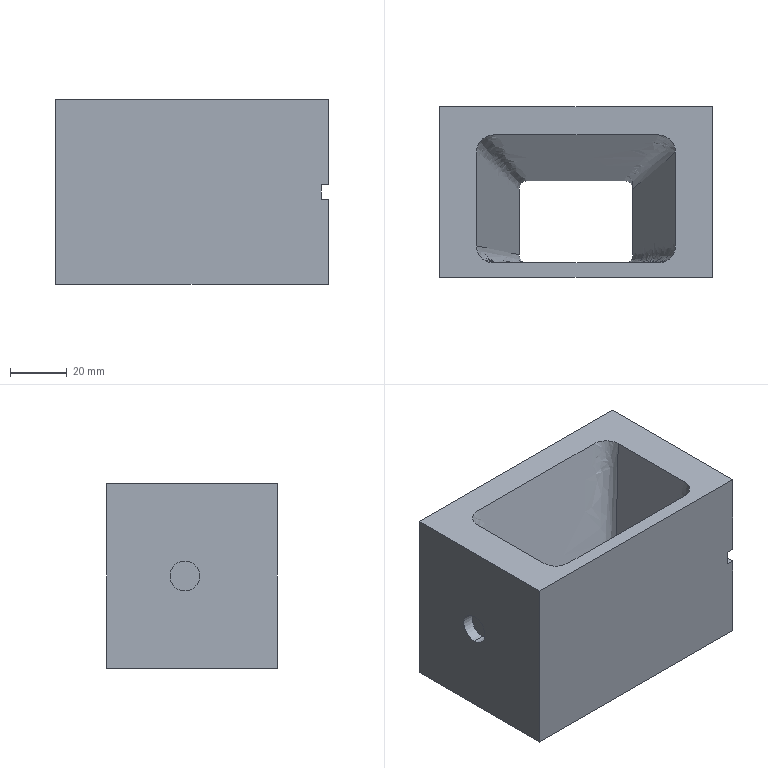Component | SolidWorks | CuttingDie-1_Mold01-1-3 | 1 solid | 15 faces | box 96 x 60 x 65 mm | volume 243310 mm3 | plane 11 | spline 2 | cylinder 2 | commonest cylinder face diameters 10.5 x2
STEP:
#1=COLOUR_RGB('',0.7922,0.8196,0.9333);
#2=FILL_AREA_STYLE_COLOUR('',#1);
#3=FILL_AREA_STYLE('',(#2));
#4=SURFACE_STYLE_FILL_AREA(#3);
#5=SURFACE_SIDE_STYLE('',(#4));
#6=SURFACE_STYLE_USAGE(.BOTH.,#5);
#7=PRESENTATION_STYLE_ASSIGNMENT((#6));
#8=CARTESIAN_POINT('',(-18.672,-11.644,44.764));
#9=VERTEX_POINT('',#8);
#10=CARTESIAN_POINT('',(-18.672,-10.345,44.764));
#11=VERTEX_POINT('',#10);
#12=CARTESIAN_POINT('',(-18.672,-10.345,44.764));
#13=DIRECTION('',(-0.,1.,0.));
#14=VECTOR('',#13,39.37);
#15=LINE('',#12,#14);
#16=EDGE_CURVE('',#9,#11,#15,.T.);
#17=ORIENTED_EDGE('',*,*,#16,.F.);
#18=CARTESIAN_POINT('',(-18.082,-11.762,42.205));
#19=VERTEX_POINT('',#18);
#20=CARTESIAN_POINT('',(-18.672,-11.644,44.764));
#21=CARTESIAN_POINT('',(-18.475,-11.684,43.911));
#22=CARTESIAN_POINT('',(-18.278,-11.723,43.058));
#23=CARTESIAN_POINT('',(-18.082,-11.762,42.205));
#24=B_SPLINE_CURVE_WITH_KNOTS('',3,(#20,#21,#22,#23),.UNSPECIFIED.,.F.,.F.,(4,4),(0.,1.),.UNSPECIFIED.);
#25=EDGE_CURVE('',#9,#19,#24,.T.);
#26=ORIENTED_EDGE('',*,*,#25,.T.);
#27=CARTESIAN_POINT('',(-18.082,-10.857,42.205));
#28=VERTEX_POINT('',#27);
#29=CARTESIAN_POINT('',(-18.082,-11.762,42.205));
#30=DIRECTION('',(0.,-1.,-0.));
#31=VECTOR('',#30,39.37);
#32=LINE('',#29,#31);
#33=EDGE_CURVE('',#28,#19,#32,.T.);
#34=ORIENTED_EDGE('',*,*,#33,.F.);
#35=CARTESIAN_POINT('',(-17.963,-10.739,42.205));
#36=VERTEX_POINT('',#35);
#37=CARTESIAN_POINT('',(-17.963,-10.857,42.205));
#38=DIRECTION('',(-0.,-0.,1.));
#39=DIRECTION('',(-1.,0.,0.));
#40=AXIS2_PLACEMENT_3D('',#37,#38,#39);
#41=CIRCLE('',#40,0.1181);
#42=EDGE_CURVE('',#36,#28,#41,.T.);
#43=ORIENTED_EDGE('',*,*,#42,.F.);
#44=CARTESIAN_POINT('',(-16.625,-10.739,42.205));
#45=VERTEX_POINT('',#44);
#46=CARTESIAN_POINT('',(-17.963,-10.739,42.205));
#47=DIRECTION('',(-1.,-0.,-0.));
#48=VECTOR('',#47,39.37);
#49=LINE('',#46,#48);
#50=EDGE_CURVE('',#45,#36,#49,.T.);
#51=ORIENTED_EDGE('',*,*,#50,.F.);
#52=CARTESIAN_POINT('',(-16.507,-10.857,42.205));
#53=VERTEX_POINT('',#52);
#54=CARTESIAN_POINT('',(-16.625,-10.857,42.205));
#55=DIRECTION('',(-0.,-0.,1.));
#56=DIRECTION('',(-1.,0.,0.));
#57=AXIS2_PLACEMENT_3D('',#54,#55,#56);
#58=CIRCLE('',#57,0.1181);
#59=EDGE_CURVE('',#53,#45,#58,.T.);
#60=ORIENTED_EDGE('',*,*,#59,.F.);
#61=CARTESIAN_POINT('',(-15.916,-10.345,44.764));
#62=VERTEX_POINT('',#61);
#63=CARTESIAN_POINT('',(-15.916,-10.345,44.764));
#64=CARTESIAN_POINT('',(-16.113,-10.516,43.911));
#65=CARTESIAN_POINT('',(-16.31,-10.686,43.058));
#66=CARTESIAN_POINT('',(-16.507,-10.857,42.205));
#67=B_SPLINE_CURVE_WITH_KNOTS('',3,(#63,#64,#65,#66),.UNSPECIFIED.,.F.,.F.,(4,4),(0.,1.),.UNSPECIFIED.);
#68=EDGE_CURVE('',#62,#53,#67,.T.);
#69=ORIENTED_EDGE('',*,*,#68,.F.);
#70=CARTESIAN_POINT('',(-16.152,-10.109,44.764));
#71=VERTEX_POINT('',#70);
#72=CARTESIAN_POINT('',(-16.152,-10.345,44.764));
#73=DIRECTION('',(0.,0.,-1.));
#74=DIRECTION('',(-1.,0.,0.));
#75=AXIS2_PLACEMENT_3D('',#72,#73,#74);
#76=CIRCLE('',#75,0.2362);
#77=EDGE_CURVE('',#71,#62,#76,.T.);
#78=ORIENTED_EDGE('',*,*,#77,.F.);
#79=CARTESIAN_POINT('',(-18.436,-10.109,44.764));
#80=VERTEX_POINT('',#79);
#81=CARTESIAN_POINT('',(-16.152,-10.109,44.764));
#82=DIRECTION('',(1.,0.,0.));
#83=VECTOR('',#82,39.37);
#84=LINE('',#81,#83);
#85=EDGE_CURVE('',#80,#71,#84,.T.);
#86=ORIENTED_EDGE('',*,*,#85,.F.);
#87=CARTESIAN_POINT('',(-18.436,-10.345,44.764));
#88=DIRECTION('',(0.,0.,-1.));
#89=DIRECTION('',(1.,0.,0.));
#90=AXIS2_PLACEMENT_3D('',#87,#88,#89);
#91=CIRCLE('',#90,0.2362);
#92=EDGE_CURVE('',#11,#80,#91,.T.);
#93=ORIENTED_EDGE('',*,*,#92,.F.);
#94=EDGE_LOOP('',(#17,#26,#34,#43,#51,#60,#69,#78,#86,#93));
#95=FACE_OUTER_BOUND('',#94,.T.);
#96=CARTESIAN_POINT('',(-15.916,-10.345,44.764));
#97=CARTESIAN_POINT('',(-16.113,-10.516,43.911));
#98=CARTESIAN_POINT('',(-16.31,-10.686,43.058));
#99=CARTESIAN_POINT('',(-16.507,-10.857,42.205));
#100=CARTESIAN_POINT('',(-15.916,-10.457,44.764));
#101=CARTESIAN_POINT('',(-16.113,-10.615,43.911));
#102=CARTESIAN_POINT('',(-16.31,-10.772,43.058));
#103=CARTESIAN_POINT('',(-16.507,-10.93,42.205));
#104=CARTESIAN_POINT('',(-15.916,-10.675,44.764));
#105=CARTESIAN_POINT('',(-16.113,-10.81,43.911));
#106=CARTESIAN_POINT('',(-16.31,-10.945,43.058));
#107=CARTESIAN_POINT('',(-16.507,-11.08,42.205));
#108=CARTESIAN_POINT('',(-15.916,-10.995,44.764));
#109=CARTESIAN_POINT('',(-16.113,-11.1,43.911));
#110=CARTESIAN_POINT('',(-16.31,-11.205,43.058));
#111=CARTESIAN_POINT('',(-16.507,-11.31,42.205));
#112=CARTESIAN_POINT('',(-15.916,-11.314,44.764));
#113=CARTESIAN_POINT('',(-16.113,-11.389,43.911));
#114=CARTESIAN_POINT('',(-16.31,-11.464,43.058));
#115=CARTESIAN_POINT('',(-16.507,-11.54,42.205));
#116=CARTESIAN_POINT('',(-15.916,-11.532,44.764));
#117=CARTESIAN_POINT('',(-16.113,-11.585,43.911));
#118=CARTESIAN_POINT('',(-16.31,-11.637,43.058));
#119=CARTESIAN_POINT('',(-16.507,-11.689,42.205));
#120=CARTESIAN_POINT('',(-15.916,-11.671,44.764));
#121=CARTESIAN_POINT('',(-16.113,-11.708,43.911));
#122=CARTESIAN_POINT('',(-16.31,-11.744,43.058));
#123=CARTESIAN_POINT('',(-16.507,-11.78,42.205));
#124=CARTESIAN_POINT('',(-15.923,-11.715,44.764));
#125=CARTESIAN_POINT('',(-16.12,-11.745,43.911));
#126=CARTESIAN_POINT('',(-16.316,-11.774,43.058));
#127=CARTESIAN_POINT('',(-16.513,-11.804,42.205));
#128=CARTESIAN_POINT('',(-15.952,-11.772,44.764));
#129=CARTESIAN_POINT('',(-16.143,-11.791,43.911));
#130=CARTESIAN_POINT('',(-16.335,-11.811,43.058));
#131=CARTESIAN_POINT('',(-16.527,-11.83,42.205));
#132=CARTESIAN_POINT('',(-15.982,-11.81,44.764));
#133=CARTESIAN_POINT('',(-16.168,-11.822,43.911));
#134=CARTESIAN_POINT('',(-16.355,-11.835,43.058));
#135=CARTESIAN_POINT('',(-16.542,-11.847,42.205));
#136=CARTESIAN_POINT('',(-16.02,-11.842,44.764));
#137=CARTESIAN_POINT('',(-16.199,-11.848,43.911));
#138=CARTESIAN_POINT('',(-16.379,-11.855,43.058));
#139=CARTESIAN_POINT('',(-16.559,-11.861,42.205));
#140=CARTESIAN_POINT('',(-16.077,-11.872,44.764));
#141=CARTESIAN_POINT('',(-16.247,-11.873,43.911));
#142=CARTESIAN_POINT('',(-16.416,-11.874,43.058));
#143=CARTESIAN_POINT('',(-16.585,-11.875,42.205));
#144=CARTESIAN_POINT('',(-16.123,-11.881,44.764));
#145=CARTESIAN_POINT('',(-16.285,-11.881,43.911));
#146=CARTESIAN_POINT('',(-16.447,-11.881,43.058));
#147=CARTESIAN_POINT('',(-16.608,-11.881,42.205));
#148=CARTESIAN_POINT('',(-16.345,-11.881,44.764));
#149=CARTESIAN_POINT('',(-16.475,-11.881,43.911));
#150=CARTESIAN_POINT('',(-16.605,-11.881,43.058));
#151=CARTESIAN_POINT('',(-16.735,-11.881,42.205));
#152=CARTESIAN_POINT('',(-16.726,-11.881,44.764));
#153=CARTESIAN_POINT('',(-16.803,-11.881,43.911));
#154=CARTESIAN_POINT('',(-16.881,-11.881,43.058));
#155=CARTESIAN_POINT('',(-16.958,-11.881,42.205));
#156=CARTESIAN_POINT('',(-17.294,-11.881,44.764));
#157=CARTESIAN_POINT('',(-17.294,-11.881,43.911));
#158=CARTESIAN_POINT('',(-17.294,-11.881,43.058));
#159=CARTESIAN_POINT('',(-17.294,-11.881,42.205));
#160=CARTESIAN_POINT('',(-17.862,-11.881,44.764));
#161=CARTESIAN_POINT('',(-17.785,-11.881,43.911));
#162=CARTESIAN_POINT('',(-17.708,-11.881,43.058));
#163=CARTESIAN_POINT('',(-17.631,-11.881,42.205));
#164=CARTESIAN_POINT('',(-18.244,-11.881,44.764));
#165=CARTESIAN_POINT('',(-18.113,-11.881,43.911));
#166=CARTESIAN_POINT('',(-17.983,-11.881,43.058));
#167=CARTESIAN_POINT('',(-17.853,-11.881,42.205));
#168=CARTESIAN_POINT('',(-18.465,-11.881,44.764));
#169=CARTESIAN_POINT('',(-18.303,-11.881,43.911));
#170=CARTESIAN_POINT('',(-18.142,-11.881,43.058));
#171=CARTESIAN_POINT('',(-17.98,-11.881,42.205));
#172=CARTESIAN_POINT('',(-18.511,-11.872,44.764));
#173=CARTESIAN_POINT('',(-18.342,-11.873,43.911));
#174=CARTESIAN_POINT('',(-18.172,-11.874,43.058));
#175=CARTESIAN_POINT('',(-18.003,-11.875,42.205));
#176=CARTESIAN_POINT('',(-18.569,-11.842,44.764));
#177=CARTESIAN_POINT('',(-18.389,-11.848,43.911));
#178=CARTESIAN_POINT('',(-18.209,-11.855,43.058));
#179=CARTESIAN_POINT('',(-18.029,-11.861,42.205));
#180=CARTESIAN_POINT('',(-18.607,-11.81,44.764));
#181=CARTESIAN_POINT('',(-18.42,-11.822,43.911));
#182=CARTESIAN_POINT('',(-18.233,-11.835,43.058));
#183=CARTESIAN_POINT('',(-18.047,-11.847,42.205));
#184=CARTESIAN_POINT('',(-18.637,-11.772,44.764));
#185=CARTESIAN_POINT('',(-18.445,-11.791,43.911));
#186=CARTESIAN_POINT('',(-18.253,-11.811,43.058));
#187=CARTESIAN_POINT('',(-18.061,-11.83,42.205));
#188=CARTESIAN_POINT('',(-18.665,-11.715,44.764));
#189=CARTESIAN_POINT('',(-18.469,-11.745,43.911));
#190=CARTESIAN_POINT('',(-18.272,-11.774,43.058));
#191=CARTESIAN_POINT('',(-18.076,-11.804,42.205));
#192=CARTESIAN_POINT('',(-18.672,-11.671,44.764));
#193=CARTESIAN_POINT('',(-18.475,-11.708,43.911));
#194=CARTESIAN_POINT('',(-18.278,-11.744,43.058));
#195=CARTESIAN_POINT('',(-18.082,-11.78,42.205));
#196=CARTESIAN_POINT('',(-18.672,-11.532,44.764));
#197=CARTESIAN_POINT('',(-18.475,-11.585,43.911));
#198=CARTESIAN_POINT('',(-18.278,-11.637,43.058));
#199=CARTESIAN_POINT('',(-18.082,-11.689,42.205));
#200=CARTESIAN_POINT('',(-18.672,-11.314,44.764));
#201=CARTESIAN_POINT('',(-18.475,-11.389,43.911));
#202=CARTESIAN_POINT('',(-18.278,-11.464,43.058));
#203=CARTESIAN_POINT('',(-18.082,-11.54,42.205));
#204=CARTESIAN_POINT('',(-18.672,-10.995,44.764));
#205=CARTESIAN_POINT('',(-18.475,-11.1,43.911));
#206=CARTESIAN_POINT('',(-18.278,-11.205,43.058));
#207=CARTESIAN_POINT('',(-18.082,-11.31,42.205));
#208=CARTESIAN_POINT('',(-18.672,-10.675,44.764));
#209=CARTESIAN_POINT('',(-18.475,-10.81,43.911));
#210=CARTESIAN_POINT('',(-18.278,-10.945,43.058));
#211=CARTESIAN_POINT('',(-18.082,-11.08,42.205));
#212=CARTESIAN_POINT('',(-18.672,-10.457,44.764));
#213=CARTESIAN_POINT('',(-18.475,-10.615,43.911));
#214=CARTESIAN_POINT('',(-18.278,-10.772,43.058));
#215=CARTESIAN_POINT('',(-18.082,-10.93,42.205));
#216=CARTESIAN_POINT('',(-18.672,-10.318,44.764));
#217=CARTESIAN_POINT('',(-18.475,-10.492,43.911));
#218=CARTESIAN_POINT('',(-18.278,-10.665,43.058));
#219=CARTESIAN_POINT('',(-18.082,-10.839,42.205));
#220=CARTESIAN_POINT('',(-18.665,-10.274,44.764));
#221=CARTESIAN_POINT('',(-18.469,-10.455,43.911));
#222=CARTESIAN_POINT('',(-18.272,-10.635,43.058));
#223=CARTESIAN_POINT('',(-18.076,-10.815,42.205));
#224=CARTESIAN_POINT('',(-18.637,-10.218,44.764));
#225=CARTESIAN_POINT('',(-18.445,-10.408,43.911));
#226=CARTESIAN_POINT('',(-18.253,-10.599,43.058));
#227=CARTESIAN_POINT('',(-18.061,-10.789,42.205));
#228=CARTESIAN_POINT('',(-18.607,-10.179,44.764));
#229=CARTESIAN_POINT('',(-18.42,-10.377,43.911));
#230=CARTESIAN_POINT('',(-18.233,-10.574,43.058));
#231=CARTESIAN_POINT('',(-18.047,-10.772,42.205));
#232=CARTESIAN_POINT('',(-18.569,-10.148,44.764));
#233=CARTESIAN_POINT('',(-18.389,-10.351,43.911));
#234=CARTESIAN_POINT('',(-18.209,-10.555,43.058));
#235=CARTESIAN_POINT('',(-18.029,-10.758,42.205));
#236=CARTESIAN_POINT('',(-18.511,-10.117,44.764));
#237=CARTESIAN_POINT('',(-18.342,-10.326,43.911));
#238=CARTESIAN_POINT('',(-18.172,-10.535,43.058));
#239=CARTESIAN_POINT('',(-18.003,-10.744,42.205));
#240=CARTESIAN_POINT('',(-18.465,-10.109,44.764));
#241=CARTESIAN_POINT('',(-18.303,-10.319,43.911));
#242=CARTESIAN_POINT('',(-18.142,-10.529,43.058));
#243=CARTESIAN_POINT('',(-17.98,-10.739,42.205));
#244=CARTESIAN_POINT('',(-18.244,-10.109,44.764));
#245=CARTESIAN_POINT('',(-18.113,-10.319,43.911));
#246=CARTESIAN_POINT('',(-17.983,-10.529,43.058));
#247=CARTESIAN_POINT('',(-17.853,-10.739,42.205));
#248=CARTESIAN_POINT('',(-17.862,-10.109,44.764));
#249=CARTESIAN_POINT('',(-17.785,-10.319,43.911));
#250=CARTESIAN_POINT('',(-17.708,-10.529,43.058));
#251=CARTESIAN_POINT('',(-17.631,-10.739,42.205));
#252=CARTESIAN_POINT('',(-17.294,-10.109,44.764));
#253=CARTESIAN_POINT('',(-17.294,-10.319,43.911));
#254=CARTESIAN_POINT('',(-17.294,-10.529,43.058));
#255=CARTESIAN_POINT('',(-17.294,-10.739,42.205));
#256=CARTESIAN_POINT('',(-16.726,-10.109,44.764));
#257=CARTESIAN_POINT('',(-16.803,-10.319,43.911));
#258=CARTESIAN_POINT('',(-16.881,-10.529,43.058));
#259=CARTESIAN_POINT('',(-16.958,-10.739,42.205));
#260=CARTESIAN_POINT('',(-16.345,-10.109,44.764));
#261=CARTESIAN_POINT('',(-16.475,-10.319,43.911));
#262=CARTESIAN_POINT('',(-16.605,-10.529,43.058));
#263=CARTESIAN_POINT('',(-16.735,-10.739,42.205));
#264=CARTESIAN_POINT('',(-16.123,-10.109,44.764));
#265=CARTESIAN_POINT('',(-16.285,-10.319,43.911));
#266=CARTESIAN_POINT('',(-16.447,-10.529,43.058));
#267=CARTESIAN_POINT('',(-16.608,-10.739,42.205));
#268=CARTESIAN_POINT('',(-16.077,-10.117,44.764));
#269=CARTESIAN_POINT('',(-16.247,-10.326,43.911));
#270=CARTESIAN_POINT('',(-16.416,-10.535,43.058));
#271=CARTESIAN_POINT('',(-16.585,-10.744,42.205));
#272=CARTESIAN_POINT('',(-16.02,-10.148,44.764));
#273=CARTESIAN_POINT('',(-16.199,-10.351,43.911));
#274=CARTESIAN_POINT('',(-16.379,-10.555,43.058));
#275=CARTESIAN_POINT('',(-16.559,-10.758,42.205));
#276=CARTESIAN_POINT('',(-15.982,-10.179,44.764));
#277=CARTESIAN_POINT('',(-16.168,-10.377,43.911));
#278=CARTESIAN_POINT('',(-16.355,-10.574,43.058));
#279=CARTESIAN_POINT('',(-16.542,-10.772,42.205));
#280=CARTESIAN_POINT('',(-15.952,-10.218,44.764));
#281=CARTESIAN_POINT('',(-16.143,-10.408,43.911));
#282=CARTESIAN_POINT('',(-16.335,-10.599,43.058));
#283=CARTESIAN_POINT('',(-16.527,-10.789,42.205));
#284=CARTESIAN_POINT('',(-15.923,-10.274,44.764));
#285=CARTESIAN_POINT('',(-16.12,-10.455,43.911));
#286=CARTESIAN_POINT('',(-16.316,-10.635,43.058));
#287=CARTESIAN_POINT('',(-16.513,-10.815,42.205));
#288=CARTESIAN_POINT('',(-15.916,-10.318,44.764));
#289=CARTESIAN_POINT('',(-16.113,-10.492,43.911));
#290=CARTESIAN_POINT('',(-16.31,-10.665,43.058));
#291=CARTESIAN_POINT('',(-16.507,-10.839,42.205));
#292=CARTESIAN_POINT('',(-15.916,-10.345,44.764));
#293=CARTESIAN_POINT('',(-16.113,-10.516,43.911));
#294=CARTESIAN_POINT('',(-16.31,-10.686,43.058));
#295=CARTESIAN_POINT('',(-16.507,-10.857,42.205));
#296=B_SPLINE_SURFACE_WITH_KNOTS('',3,3,((#96,#97,#98,#99),(#100,#101,#102,#103),(#104,#105,#106,#107),(#108,#109,#110,#111),(#112,#113,#114,#115),(#116,#117,#118,#119),(#120,#121,#122,#123),(#124,#125,#126,#127),(#128,#129,#130,#131),(#132,#133,#134,#135),(#136,#137,#138,#139),(#140,#141,#142,#143),(#144,#145,#146,#147),(#148,#149,#150,#151),(#152,#153,#154,#155),(#156,#157,#158,#159),(#160,#161,#162,#163),(#164,#165,#166,#167),(#168,#169,#170,#171),(#172,#173,#174,#175),(#176,#177,#178,#179),(#180,#181,#182,#183),(#184,#185,#186,#187),(#188,#189,#190,#191),(#192,#193,#194,#195),(#196,#197,#198,#199),(#200,#201,#202,#203),(#204,#205,#206,#207),(#208,#209,#210,#211),(#212,#213,#214,#215),(#216,#217,#218,#219),(#220,#221,#222,#223),(#224,#225,#226,#227),(#228,#229,#230,#231),(#232,#233,#234,#235),(#236,#237,#238,#239),(#240,#241,#242,#243),(#244,#245,#246,#247),(#248,#249,#250,#251),(#252,#253,#254,#255),(#256,#257,#258,#259),(#260,#261,#262,#263),(#264,#265,#266,#267),(#268,#269,#270,#271),(#272,#273,#274,#275),(#276,#277,#278,#279),(#280,#281,#282,#283),(#284,#285,#286,#287),(#288,#289,#290,#291),(#292,#293,#294,#295)),.UNSPECIFIED.,.T.,.F.,.F.,(4,1,1,1,2,1,1,1,1,1,2,1,1,1,2,1,1,1,1,1,2,1,1,1,2,1,1,1,1,1,2,1,1,1,2,1,1,1,1,1,4),(4,4),(0.,0.04042,0.08083,0.1213,0.1617,0.1715,0.1764,0.1813,0.1862,0.1911,0.2009,0.2658,0.3308,0.3958,0.4608,0.4706,0.4755,0.4804,0.4853,0.4902,0.5,0.5404,0.5808,0.6213,0.6617,0.6715,0.6764,0.6813,0.6862,0.6911,0.7009,0.7658,0.8308,0.8958,0.9608,0.9706,0.9755,0.9804,0.9853,0.9902,1.),(0.,1.),.UNSPECIFIED.);
#297=ADVANCED_FACE('',(#95),#296,.F.);
#298=CARTESIAN_POINT('',(-19.026,-10.798,43.278));
#299=VERTEX_POINT('',#298);
#300=CARTESIAN_POINT('',(-19.026,-10.798,43.691));
#301=VERTEX_POINT('',#300);
#302=CARTESIAN_POINT('',(-19.026,-10.798,43.484));
#303=DIRECTION('',(-1.,-0.,-0.));
#304=DIRECTION('',(0.,0.,1.));
#305=AXIS2_PLACEMENT_3D('',#302,#303,#304);
#306=CIRCLE('',#305,0.2067);
#307=EDGE_CURVE('',#299,#301,#306,.T.);
#308=ORIENTED_EDGE('',*,*,#307,.F.);
#309=CARTESIAN_POINT('',(-19.184,-10.798,43.278));
#310=VERTEX_POINT('',#309);
#311=CARTESIAN_POINT('',(-19.026,-10.798,43.278));
#312=DIRECTION('',(-1.,-0.,-0.));
#313=VECTOR('',#312,39.37);
#314=LINE('',#311,#313);
#315=EDGE_CURVE('',#299,#310,#314,.T.);
#316=ORIENTED_EDGE('',*,*,#315,.T.);
#317=CARTESIAN_POINT('',(-19.184,-10.798,43.691));
#318=VERTEX_POINT('',#317);
#319=CARTESIAN_POINT('',(-19.184,-10.798,43.484));
#320=DIRECTION('',(-1.,-0.,-0.));
#321=DIRECTION('',(0.,0.,1.));
#322=AXIS2_PLACEMENT_3D('',#319,#320,#321);
#323=CIRCLE('',#322,0.2067);
#324=EDGE_CURVE('',#310,#318,#323,.T.);
#325=ORIENTED_EDGE('',*,*,#324,.T.);
#326=CARTESIAN_POINT('',(-19.026,-10.798,43.691));
#327=DIRECTION('',(-1.,-0.,-0.));
#328=VECTOR('',#327,39.37);
#329=LINE('',#326,#328);
#330=EDGE_CURVE('',#301,#318,#329,.T.);
#331=ORIENTED_EDGE('',*,*,#330,.F.);
#332=EDGE_LOOP('',(#308,#316,#325,#331));
#333=FACE_OUTER_BOUND('',#332,.T.);
#334=CARTESIAN_POINT('',(-19.026,-10.798,43.484));
#335=DIRECTION('',(-1.,-0.,-0.));
#336=DIRECTION('',(0.,0.,1.));
#337=AXIS2_PLACEMENT_3D('',#334,#335,#336);
#338=CYLINDRICAL_SURFACE('',#337,0.2067);
#339=ADVANCED_FACE('',(#333),#338,.F.);
#340=CARTESIAN_POINT('',(-15.404,-9.715,42.205));
#341=VERTEX_POINT('',#340);
#342=CARTESIAN_POINT('',(-15.404,-12.077,42.205));
#343=VERTEX_POINT('',#342);
#344=CARTESIAN_POINT('',(-15.404,-9.518,42.205));
#345=DIRECTION('',(0.,-1.,-0.));
#346=VECTOR('',#345,39.37);
#347=LINE('',#344,#346);
#348=EDGE_CURVE('',#341,#343,#347,.T.);
#349=ORIENTED_EDGE('',*,*,#348,.F.);
#350=CARTESIAN_POINT('',(-15.404,-9.715,43.386));
#351=VERTEX_POINT('',#350);
#352=CARTESIAN_POINT('',(-15.404,-9.715,42.205));
#353=DIRECTION('',(-0.,-0.,1.));
#354=VECTOR('',#353,39.37);
#355=LINE('',#352,#354);
#356=EDGE_CURVE('',#341,#351,#355,.T.);
#357=ORIENTED_EDGE('',*,*,#356,.T.);
#358=CARTESIAN_POINT('',(-15.404,-12.077,43.386));
#359=VERTEX_POINT('',#358);
#360=CARTESIAN_POINT('',(-15.404,-12.077,43.386));
#361=DIRECTION('',(-0.,1.,0.));
#362=VECTOR('',#361,39.37);
#363=LINE('',#360,#362);
#364=EDGE_CURVE('',#359,#351,#363,.T.);
#365=ORIENTED_EDGE('',*,*,#364,.F.);
#366=CARTESIAN_POINT('',(-15.404,-12.077,42.205));
#367=DIRECTION('',(0.,0.,-1.));
#368=VECTOR('',#367,39.37);
#369=LINE('',#366,#368);
#370=EDGE_CURVE('',#359,#343,#369,.T.);
#371=ORIENTED_EDGE('',*,*,#370,.T.);
#372=EDGE_LOOP('',(#349,#357,#365,#371));
#373=FACE_OUTER_BOUND('',#372,.T.);
#374=CARTESIAN_POINT('',(-15.404,-9.518,42.205));
#375=DIRECTION('',(-1.,-0.,-0.));
#376=DIRECTION('',(-0.,-0.,1.));
#377=AXIS2_PLACEMENT_3D('',#374,#375,#376);
#378=PLANE('',#377);
#379=ADVANCED_FACE('',(#373),#378,.F.);
#380=ORIENTED_EDGE('',*,*,#77,.T.);
#381=CARTESIAN_POINT('',(-15.916,-11.644,44.764));
#382=VERTEX_POINT('',#381);
#383=CARTESIAN_POINT('',(-15.916,-10.345,44.764));
#384=DIRECTION('',(-0.,-1.,-0.));
#385=VECTOR('',#384,39.37);
#386=LINE('',#383,#385);
#387=EDGE_CURVE('',#62,#382,#386,.T.);
#388=ORIENTED_EDGE('',*,*,#387,.T.);
#389=CARTESIAN_POINT('',(-16.152,-11.881,44.764));
#390=VERTEX_POINT('',#389);
#391=CARTESIAN_POINT('',(-16.152,-11.644,44.764));
#392=DIRECTION('',(0.,0.,-1.));
#393=DIRECTION('',(-1.,0.,0.));
#394=AXIS2_PLACEMENT_3D('',#391,#392,#393);
#395=CIRCLE('',#394,0.2362);
#396=EDGE_CURVE('',#382,#390,#395,.T.);
#397=ORIENTED_EDGE('',*,*,#396,.T.);
#398=CARTESIAN_POINT('',(-18.436,-11.881,44.764));
#399=VERTEX_POINT('',#398);
#400=CARTESIAN_POINT('',(-16.152,-11.881,44.764));
#401=DIRECTION('',(-1.,-0.,-0.));
#402=VECTOR('',#401,39.37);
#403=LINE('',#400,#402);
#404=EDGE_CURVE('',#390,#399,#403,.T.);
#405=ORIENTED_EDGE('',*,*,#404,.T.);
#406=CARTESIAN_POINT('',(-18.436,-11.644,44.764));
#407=DIRECTION('',(0.,0.,-1.));
#408=DIRECTION('',(-1.,0.,0.));
#409=AXIS2_PLACEMENT_3D('',#406,#407,#408);
#410=CIRCLE('',#409,0.2362);
#411=EDGE_CURVE('',#399,#9,#410,.T.);
#412=ORIENTED_EDGE('',*,*,#411,.T.);
#413=ORIENTED_EDGE('',*,*,#16,.T.);
#414=ORIENTED_EDGE('',*,*,#92,.T.);
#415=ORIENTED_EDGE('',*,*,#85,.T.);
#416=EDGE_LOOP('',(#380,#388,#397,#405,#412,#413,#414,#415));
#417=FACE_BOUND('',#416,.T.);
#418=CARTESIAN_POINT('',(-15.404,-9.715,44.764));
#419=VERTEX_POINT('',#418);
#420=CARTESIAN_POINT('',(-15.404,-12.077,44.764));
#421=VERTEX_POINT('',#420);
#422=CARTESIAN_POINT('',(-15.404,-9.518,44.764));
#423=DIRECTION('',(0.,-1.,-0.));
#424=VECTOR('',#423,39.37);
#425=LINE('',#422,#424);
#426=EDGE_CURVE('',#419,#421,#425,.T.);
#427=ORIENTED_EDGE('',*,*,#426,.F.);
#428=CARTESIAN_POINT('',(-19.184,-9.715,44.764));
#429=VERTEX_POINT('',#428);
#430=CARTESIAN_POINT('',(-15.404,-9.715,44.764));
#431=DIRECTION('',(-1.,-0.,-0.));
#432=VECTOR('',#431,39.37);
#433=LINE('',#430,#432);
#434=EDGE_CURVE('',#419,#429,#433,.T.);
#435=ORIENTED_EDGE('',*,*,#434,.T.);
#436=CARTESIAN_POINT('',(-19.184,-12.077,44.764));
#437=VERTEX_POINT('',#436);
#438=CARTESIAN_POINT('',(-19.184,-9.518,44.764));
#439=DIRECTION('',(0.,-1.,-0.));
#440=VECTOR('',#439,39.37);
#441=LINE('',#438,#440);
#442=EDGE_CURVE('',#429,#437,#441,.T.);
#443=ORIENTED_EDGE('',*,*,#442,.T.);
#444=CARTESIAN_POINT('',(-19.184,-12.077,44.764));
#445=DIRECTION('',(1.,0.,0.));
#446=VECTOR('',#445,39.37);
#447=LINE('',#444,#446);
#448=EDGE_CURVE('',#437,#421,#447,.T.);
#449=ORIENTED_EDGE('',*,*,#448,.T.);
#450=EDGE_LOOP('',(#427,#435,#443,#449));
#451=FACE_OUTER_BOUND('',#450,.T.);
#452=CARTESIAN_POINT('',(-19.184,-9.518,44.764));
#453=DIRECTION('',(0.,0.,-1.));
#454=DIRECTION('',(-1.,-0.,-0.));
#455=AXIS2_PLACEMENT_3D('',#452,#453,#454);
#456=PLANE('',#455);
#457=ADVANCED_FACE('',(#417,#451),#456,.F.);
#458=CARTESIAN_POINT('',(-15.404,-12.077,43.583));
#459=VERTEX_POINT('',#458);
#460=CARTESIAN_POINT('',(-15.404,-9.715,43.583));
#461=VERTEX_POINT('',#460);
#462=CARTESIAN_POINT('',(-15.404,-12.077,43.583));
#463=DIRECTION('',(-0.,1.,0.));
#464=VECTOR('',#463,39.37);
#465=LINE('',#462,#464);
#466=EDGE_CURVE('',#459,#461,#465,.T.);
#467=ORIENTED_EDGE('',*,*,#466,.T.);
#468=CARTESIAN_POINT('',(-15.404,-9.715,42.205));
#469=DIRECTION('',(-0.,-0.,1.));
#470=VECTOR('',#469,39.37);
#471=LINE('',#468,#470);
#472=EDGE_CURVE('',#461,#419,#471,.T.);
#473=ORIENTED_EDGE('',*,*,#472,.T.);
#474=ORIENTED_EDGE('',*,*,#426,.T.);
#475=CARTESIAN_POINT('',(-15.404,-12.077,42.205));
#476=DIRECTION('',(0.,0.,-1.));
#477=VECTOR('',#476,39.37);
#478=LINE('',#475,#477);
#479=EDGE_CURVE('',#421,#459,#478,.T.);
#480=ORIENTED_EDGE('',*,*,#479,.T.);
#481=EDGE_LOOP('',(#467,#473,#474,#480));
#482=FACE_OUTER_BOUND('',#481,.T.);
#483=CARTESIAN_POINT('',(-15.404,-9.518,42.205));
#484=DIRECTION('',(-1.,-0.,-0.));
#485=DIRECTION('',(-0.,-0.,1.));
#486=AXIS2_PLACEMENT_3D('',#483,#484,#485);
#487=PLANE('',#486);
#488=ADVANCED_FACE('',(#482),#487,.F.);
#489=CARTESIAN_POINT('',(-16.507,-11.762,42.205));
#490=VERTEX_POINT('',#489);
#491=CARTESIAN_POINT('',(-16.507,-11.762,42.205));
#492=DIRECTION('',(-0.,1.,0.));
#493=VECTOR('',#492,39.37);
#494=LINE('',#491,#493);
#495=EDGE_CURVE('',#490,#53,#494,.T.);
#496=ORIENTED_EDGE('',*,*,#495,.T.);
#497=ORIENTED_EDGE('',*,*,#59,.T.);
#498=ORIENTED_EDGE('',*,*,#50,.T.);
#499=ORIENTED_EDGE('',*,*,#42,.T.);
#500=ORIENTED_EDGE('',*,*,#33,.T.);
#501=CARTESIAN_POINT('',(-17.963,-11.881,42.205));
#502=VERTEX_POINT('',#501);
#503=CARTESIAN_POINT('',(-17.963,-11.762,42.205));
#504=DIRECTION('',(-0.,-0.,1.));
#505=DIRECTION('',(-1.,0.,0.));
#506=AXIS2_PLACEMENT_3D('',#503,#504,#505);
#507=CIRCLE('',#506,0.1181);
#508=EDGE_CURVE('',#19,#502,#507,.T.);
#509=ORIENTED_EDGE('',*,*,#508,.T.);
#510=CARTESIAN_POINT('',(-16.625,-11.881,42.205));
#511=VERTEX_POINT('',#510);
#512=CARTESIAN_POINT('',(-17.963,-11.881,42.205));
#513=DIRECTION('',(1.,0.,0.));
#514=VECTOR('',#513,39.37);
#515=LINE('',#512,#514);
#516=EDGE_CURVE('',#502,#511,#515,.T.);
#517=ORIENTED_EDGE('',*,*,#516,.T.);
#518=CARTESIAN_POINT('',(-16.625,-11.762,42.205));
#519=DIRECTION('',(-0.,-0.,1.));
#520=DIRECTION('',(1.,0.,0.));
#521=AXIS2_PLACEMENT_3D('',#518,#519,#520);
#522=CIRCLE('',#521,0.1181);
#523=EDGE_CURVE('',#511,#490,#522,.T.);
#524=ORIENTED_EDGE('',*,*,#523,.T.);
#525=EDGE_LOOP('',(#496,#497,#498,#499,#500,#509,#517,#524));
#526=FACE_BOUND('',#525,.T.);
#527=CARTESIAN_POINT('',(-19.184,-9.715,42.205));
#528=VERTEX_POINT('',#527);
#529=CARTESIAN_POINT('',(-19.184,-12.077,42.205));
#530=VERTEX_POINT('',#529);
#531=CARTESIAN_POINT('',(-19.184,-9.518,42.205));
#532=DIRECTION('',(0.,-1.,-0.));
#533=VECTOR('',#532,39.37);
#534=LINE('',#531,#533);
#535=EDGE_CURVE('',#528,#530,#534,.T.);
#536=ORIENTED_EDGE('',*,*,#535,.F.);
#537=CARTESIAN_POINT('',(-15.404,-9.715,42.205));
#538=DIRECTION('',(-1.,-0.,-0.));
#539=VECTOR('',#538,39.37);
#540=LINE('',#537,#539);
#541=EDGE_CURVE('',#341,#528,#540,.T.);
#542=ORIENTED_EDGE('',*,*,#541,.F.);
#543=ORIENTED_EDGE('',*,*,#348,.T.);
#544=CARTESIAN_POINT('',(-19.184,-12.077,42.205));
#545=DIRECTION('',(-1.,-0.,-0.));
#546=VECTOR('',#545,39.37);
#547=LINE('',#544,#546);
#548=EDGE_CURVE('',#343,#530,#547,.T.);
#549=ORIENTED_EDGE('',*,*,#548,.T.);
#550=EDGE_LOOP('',(#536,#542,#543,#549));
#551=FACE_OUTER_BOUND('',#550,.T.);
#552=CARTESIAN_POINT('',(-19.184,-9.518,42.205));
#553=DIRECTION('',(-0.,-0.,1.));
#554=DIRECTION('',(1.,0.,0.));
#555=AXIS2_PLACEMENT_3D('',#552,#553,#554);
#556=PLANE('',#555);
#557=ADVANCED_FACE('',(#526,#551),#556,.F.);
#558=CARTESIAN_POINT('',(-19.184,-10.798,43.484));
#559=DIRECTION('',(-1.,-0.,-0.));
#560=DIRECTION('',(0.,0.,1.));
#561=AXIS2_PLACEMENT_3D('',#558,#559,#560);
#562=CIRCLE('',#561,0.2067);
#563=EDGE_CURVE('',#318,#310,#562,.T.);
#564=ORIENTED_EDGE('',*,*,#563,.F.);
#565=ORIENTED_EDGE('',*,*,#324,.F.);
#566=EDGE_LOOP('',(#564,#565));
#567=FACE_BOUND('',#566,.T.);
#568=ORIENTED_EDGE('',*,*,#442,.F.);
#569=CARTESIAN_POINT('',(-19.184,-9.715,42.205));
#570=DIRECTION('',(-0.,-0.,1.));
#571=VECTOR('',#570,39.37);
#572=LINE('',#569,#571);
#573=EDGE_CURVE('',#528,#429,#572,.T.);
#574=ORIENTED_EDGE('',*,*,#573,.F.);
#575=ORIENTED_EDGE('',*,*,#535,.T.);
#576=CARTESIAN_POINT('',(-19.184,-12.077,42.205));
#577=DIRECTION('',(-0.,-0.,1.));
#578=VECTOR('',#577,39.37);
#579=LINE('',#576,#578);
#580=EDGE_CURVE('',#530,#437,#579,.T.);
#581=ORIENTED_EDGE('',*,*,#580,.T.);
#582=EDGE_LOOP('',(#568,#574,#575,#581));
#583=FACE_OUTER_BOUND('',#582,.T.);
#584=CARTESIAN_POINT('',(-19.184,-9.518,42.205));
#585=DIRECTION('',(1.,0.,0.));
#586=DIRECTION('',(0.,0.,-1.));
#587=AXIS2_PLACEMENT_3D('',#584,#585,#586);
#588=PLANE('',#587);
#589=ADVANCED_FACE('',(#567,#583),#588,.F.);
#590=CARTESIAN_POINT('',(-15.503,-12.077,43.386));
#591=VERTEX_POINT('',#590);
#592=CARTESIAN_POINT('',(-15.404,-12.077,43.386));
#593=DIRECTION('',(-1.,-0.,-0.));
#594=VECTOR('',#593,39.37);
#595=LINE('',#592,#594);
#596=EDGE_CURVE('',#359,#591,#595,.T.);
#597=ORIENTED_EDGE('',*,*,#596,.T.);
#598=CARTESIAN_POINT('',(-15.503,-12.077,43.583));
#599=VERTEX_POINT('',#598);
#600=CARTESIAN_POINT('',(-15.503,-12.077,43.386));
#601=DIRECTION('',(-0.,-0.,1.));
#602=VECTOR('',#601,39.37);
#603=LINE('',#600,#602);
#604=EDGE_CURVE('',#591,#599,#603,.T.);
#605=ORIENTED_EDGE('',*,*,#604,.T.);
#606=CARTESIAN_POINT('',(-15.404,-12.077,43.583));
#607=DIRECTION('',(1.,0.,0.));
#608=VECTOR('',#607,39.37);
#609=LINE('',#606,#608);
#610=EDGE_CURVE('',#599,#459,#609,.T.);
#611=ORIENTED_EDGE('',*,*,#610,.T.);
#612=ORIENTED_EDGE('',*,*,#479,.F.);
#613=ORIENTED_EDGE('',*,*,#448,.F.);
#614=ORIENTED_EDGE('',*,*,#580,.F.);
#615=ORIENTED_EDGE('',*,*,#548,.F.);
#616=ORIENTED_EDGE('',*,*,#370,.F.);
#617=EDGE_LOOP('',(#597,#605,#611,#612,#613,#614,#615,#616));
#618=FACE_OUTER_BOUND('',#617,.T.);
#619=CARTESIAN_POINT('',(-17.294,-12.077,43.484));
#620=DIRECTION('',(0.,-1.,-0.));
#621=DIRECTION('',(1.,0.,0.));
#622=AXIS2_PLACEMENT_3D('',#619,#620,#621);
#623=PLANE('',#622);
#624=ADVANCED_FACE('',(#618),#623,.T.);
#625=ORIENTED_EDGE('',*,*,#364,.T.);
#626=CARTESIAN_POINT('',(-15.503,-9.715,43.386));
#627=VERTEX_POINT('',#626);
#628=CARTESIAN_POINT('',(-15.404,-9.715,43.386));
#629=DIRECTION('',(-1.,-0.,-0.));
#630=VECTOR('',#629,39.37);
#631=LINE('',#628,#630);
#632=EDGE_CURVE('',#351,#627,#631,.T.);
#633=ORIENTED_EDGE('',*,*,#632,.T.);
#634=CARTESIAN_POINT('',(-15.503,-12.077,43.386));
#635=DIRECTION('',(-0.,1.,0.));
#636=VECTOR('',#635,39.37);
#637=LINE('',#634,#636);
#638=EDGE_CURVE('',#591,#627,#637,.T.);
#639=ORIENTED_EDGE('',*,*,#638,.F.);
#640=ORIENTED_EDGE('',*,*,#596,.F.);
#641=EDGE_LOOP('',(#625,#633,#639,#640));
#642=FACE_OUTER_BOUND('',#641,.T.);
#643=CARTESIAN_POINT('',(-15.404,-12.077,43.386));
#644=DIRECTION('',(0.,0.,-1.));
#645=DIRECTION('',(-1.,-0.,-0.));
#646=AXIS2_PLACEMENT_3D('',#643,#644,#645);
#647=PLANE('',#646);
#648=ADVANCED_FACE('',(#642),#647,.F.);
#649=CARTESIAN_POINT('',(-15.503,-9.715,43.583));
#650=VERTEX_POINT('',#649);
#651=CARTESIAN_POINT('',(-15.503,-12.077,43.583));
#652=DIRECTION('',(-0.,1.,0.));
#653=VECTOR('',#652,39.37);
#654=LINE('',#651,#653);
#655=EDGE_CURVE('',#599,#650,#654,.T.);
#656=ORIENTED_EDGE('',*,*,#655,.T.);
#657=CARTESIAN_POINT('',(-15.404,-9.715,43.583));
#658=DIRECTION('',(1.,0.,0.));
#659=VECTOR('',#658,39.37);
#660=LINE('',#657,#659);
#661=EDGE_CURVE('',#650,#461,#660,.T.);
#662=ORIENTED_EDGE('',*,*,#661,.T.);
#663=ORIENTED_EDGE('',*,*,#466,.F.);
#664=ORIENTED_EDGE('',*,*,#610,.F.);
#665=EDGE_LOOP('',(#656,#662,#663,#664));
#666=FACE_OUTER_BOUND('',#665,.T.);
#667=CARTESIAN_POINT('',(-15.404,-12.077,43.583));
#668=DIRECTION('',(-0.,-0.,1.));
#669=DIRECTION('',(1.,0.,0.));
#670=AXIS2_PLACEMENT_3D('',#667,#668,#669);
#671=PLANE('',#670);
#672=ADVANCED_FACE('',(#666),#671,.F.);
#673=ORIENTED_EDGE('',*,*,#638,.T.);
#674=CARTESIAN_POINT('',(-15.503,-9.715,43.386));
#675=DIRECTION('',(-0.,-0.,1.));
#676=VECTOR('',#675,39.37);
#677=LINE('',#674,#676);
#678=EDGE_CURVE('',#627,#650,#677,.T.);
#679=ORIENTED_EDGE('',*,*,#678,.T.);
#680=ORIENTED_EDGE('',*,*,#655,.F.);
#681=ORIENTED_EDGE('',*,*,#604,.F.);
#682=EDGE_LOOP('',(#673,#679,#680,#681));
#683=FACE_OUTER_BOUND('',#682,.T.);
#684=CARTESIAN_POINT('',(-15.503,-12.077,43.386));
#685=DIRECTION('',(-1.,-0.,-0.));
#686=DIRECTION('',(-0.,-0.,1.));
#687=AXIS2_PLACEMENT_3D('',#684,#685,#686);
#688=PLANE('',#687);
#689=ADVANCED_FACE('',(#683),#688,.F.);
#690=ORIENTED_EDGE('',*,*,#315,.F.);
#691=CARTESIAN_POINT('',(-19.026,-10.798,43.484));
#692=DIRECTION('',(-1.,-0.,-0.));
#693=DIRECTION('',(0.,0.,1.));
#694=AXIS2_PLACEMENT_3D('',#691,#692,#693);
#695=CIRCLE('',#694,0.2067);
#696=EDGE_CURVE('',#301,#299,#695,.T.);
#697=ORIENTED_EDGE('',*,*,#696,.F.);
#698=ORIENTED_EDGE('',*,*,#330,.T.);
#699=ORIENTED_EDGE('',*,*,#563,.T.);
#700=EDGE_LOOP('',(#690,#697,#698,#699));
#701=FACE_OUTER_BOUND('',#700,.T.);
#702=CARTESIAN_POINT('',(-19.026,-10.798,43.484));
#703=DIRECTION('',(-1.,-0.,-0.));
#704=DIRECTION('',(0.,0.,1.));
#705=AXIS2_PLACEMENT_3D('',#702,#703,#704);
#706=CYLINDRICAL_SURFACE('',#705,0.2067);
#707=ADVANCED_FACE('',(#701),#706,.F.);
#708=ORIENTED_EDGE('',*,*,#696,.T.);
#709=ORIENTED_EDGE('',*,*,#307,.T.);
#710=EDGE_LOOP('',(#708,#709));
#711=FACE_OUTER_BOUND('',#710,.T.);
#712=CARTESIAN_POINT('',(-19.026,-10.798,43.484));
#713=DIRECTION('',(-1.,-0.,-0.));
#714=DIRECTION('',(-0.,-0.,1.));
#715=AXIS2_PLACEMENT_3D('',#712,#713,#714);
#716=PLANE('',#715);
#717=ADVANCED_FACE('',(#711),#716,.T.);
#718=ORIENTED_EDGE('',*,*,#356,.F.);
#719=ORIENTED_EDGE('',*,*,#541,.T.);
#720=ORIENTED_EDGE('',*,*,#573,.T.);
#721=ORIENTED_EDGE('',*,*,#434,.F.);
#722=ORIENTED_EDGE('',*,*,#472,.F.);
#723=ORIENTED_EDGE('',*,*,#661,.F.);
#724=ORIENTED_EDGE('',*,*,#678,.F.);
#725=ORIENTED_EDGE('',*,*,#632,.F.);
#726=EDGE_LOOP('',(#718,#719,#720,#721,#722,#723,#724,#725));
#727=FACE_OUTER_BOUND('',#726,.T.);
#728=CARTESIAN_POINT('',(-15.404,-9.715,42.205));
#729=DIRECTION('',(0.,-1.,-0.));
#730=DIRECTION('',(1.,0.,0.));
#731=AXIS2_PLACEMENT_3D('',#728,#729,#730);
#732=PLANE('',#731);
#733=ADVANCED_FACE('',(#727),#732,.F.);
#734=ORIENTED_EDGE('',*,*,#25,.F.);
#735=ORIENTED_EDGE('',*,*,#411,.F.);
#736=ORIENTED_EDGE('',*,*,#404,.F.);
#737=ORIENTED_EDGE('',*,*,#396,.F.);
#738=ORIENTED_EDGE('',*,*,#387,.F.);
#739=ORIENTED_EDGE('',*,*,#68,.T.);
#740=ORIENTED_EDGE('',*,*,#495,.F.);
#741=ORIENTED_EDGE('',*,*,#523,.F.);
#742=ORIENTED_EDGE('',*,*,#516,.F.);
#743=ORIENTED_EDGE('',*,*,#508,.F.);
#744=EDGE_LOOP('',(#734,#735,#736,#737,#738,#739,#740,#741,#742,#743));
#745=FACE_OUTER_BOUND('',#744,.T.);
#746=CARTESIAN_POINT('',(-15.916,-10.345,44.764));
#747=CARTESIAN_POINT('',(-16.113,-10.516,43.911));
#748=CARTESIAN_POINT('',(-16.31,-10.686,43.058));
#749=CARTESIAN_POINT('',(-16.507,-10.857,42.205));
#750=CARTESIAN_POINT('',(-15.916,-10.457,44.764));
#751=CARTESIAN_POINT('',(-16.113,-10.615,43.911));
#752=CARTESIAN_POINT('',(-16.31,-10.772,43.058));
#753=CARTESIAN_POINT('',(-16.507,-10.93,42.205));
#754=CARTESIAN_POINT('',(-15.916,-10.675,44.764));
#755=CARTESIAN_POINT('',(-16.113,-10.81,43.911));
#756=CARTESIAN_POINT('',(-16.31,-10.945,43.058));
#757=CARTESIAN_POINT('',(-16.507,-11.08,42.205));
#758=CARTESIAN_POINT('',(-15.916,-10.995,44.764));
#759=CARTESIAN_POINT('',(-16.113,-11.1,43.911));
#760=CARTESIAN_POINT('',(-16.31,-11.205,43.058));
#761=CARTESIAN_POINT('',(-16.507,-11.31,42.205));
#762=CARTESIAN_POINT('',(-15.916,-11.314,44.764));
#763=CARTESIAN_POINT('',(-16.113,-11.389,43.911));
#764=CARTESIAN_POINT('',(-16.31,-11.464,43.058));
#765=CARTESIAN_POINT('',(-16.507,-11.54,42.205));
#766=CARTESIAN_POINT('',(-15.916,-11.532,44.764));
#767=CARTESIAN_POINT('',(-16.113,-11.585,43.911));
#768=CARTESIAN_POINT('',(-16.31,-11.637,43.058));
#769=CARTESIAN_POINT('',(-16.507,-11.689,42.205));
#770=CARTESIAN_POINT('',(-15.916,-11.671,44.764));
#771=CARTESIAN_POINT('',(-16.113,-11.708,43.911));
#772=CARTESIAN_POINT('',(-16.31,-11.744,43.058));
#773=CARTESIAN_POINT('',(-16.507,-11.78,42.205));
#774=CARTESIAN_POINT('',(-15.923,-11.715,44.764));
#775=CARTESIAN_POINT('',(-16.12,-11.745,43.911));
#776=CARTESIAN_POINT('',(-16.316,-11.774,43.058));
#777=CARTESIAN_POINT('',(-16.513,-11.804,42.205));
#778=CARTESIAN_POINT('',(-15.952,-11.772,44.764));
#779=CARTESIAN_POINT('',(-16.143,-11.791,43.911));
#780=CARTESIAN_POINT('',(-16.335,-11.811,43.058));
#781=CARTESIAN_POINT('',(-16.527,-11.83,42.205));
#782=CARTESIAN_POINT('',(-15.982,-11.81,44.764));
#783=CARTESIAN_POINT('',(-16.168,-11.822,43.911));
#784=CARTESIAN_POINT('',(-16.355,-11.835,43.058));
#785=CARTESIAN_POINT('',(-16.542,-11.847,42.205));
#786=CARTESIAN_POINT('',(-16.02,-11.842,44.764));
#787=CARTESIAN_POINT('',(-16.199,-11.848,43.911));
#788=CARTESIAN_POINT('',(-16.379,-11.855,43.058));
#789=CARTESIAN_POINT('',(-16.559,-11.861,42.205));
#790=CARTESIAN_POINT('',(-16.077,-11.872,44.764));
#791=CARTESIAN_POINT('',(-16.247,-11.873,43.911));
#792=CARTESIAN_POINT('',(-16.416,-11.874,43.058));
#793=CARTESIAN_POINT('',(-16.585,-11.875,42.205));
#794=CARTESIAN_POINT('',(-16.123,-11.881,44.764));
#795=CARTESIAN_POINT('',(-16.285,-11.881,43.911));
#796=CARTESIAN_POINT('',(-16.447,-11.881,43.058));
#797=CARTESIAN_POINT('',(-16.608,-11.881,42.205));
#798=CARTESIAN_POINT('',(-16.345,-11.881,44.764));
#799=CARTESIAN_POINT('',(-16.475,-11.881,43.911));
#800=CARTESIAN_POINT('',(-16.605,-11.881,43.058));
#801=CARTESIAN_POINT('',(-16.735,-11.881,42.205));
#802=CARTESIAN_POINT('',(-16.726,-11.881,44.764));
#803=CARTESIAN_POINT('',(-16.803,-11.881,43.911));
#804=CARTESIAN_POINT('',(-16.881,-11.881,43.058));
#805=CARTESIAN_POINT('',(-16.958,-11.881,42.205));
#806=CARTESIAN_POINT('',(-17.294,-11.881,44.764));
#807=CARTESIAN_POINT('',(-17.294,-11.881,43.911));
#808=CARTESIAN_POINT('',(-17.294,-11.881,43.058));
#809=CARTESIAN_POINT('',(-17.294,-11.881,42.205));
#810=CARTESIAN_POINT('',(-17.862,-11.881,44.764));
#811=CARTESIAN_POINT('',(-17.785,-11.881,43.911));
#812=CARTESIAN_POINT('',(-17.708,-11.881,43.058));
#813=CARTESIAN_POINT('',(-17.631,-11.881,42.205));
#814=CARTESIAN_POINT('',(-18.244,-11.881,44.764));
#815=CARTESIAN_POINT('',(-18.113,-11.881,43.911));
#816=CARTESIAN_POINT('',(-17.983,-11.881,43.058));
#817=CARTESIAN_POINT('',(-17.853,-11.881,42.205));
#818=CARTESIAN_POINT('',(-18.465,-11.881,44.764));
#819=CARTESIAN_POINT('',(-18.303,-11.881,43.911));
#820=CARTESIAN_POINT('',(-18.142,-11.881,43.058));
#821=CARTESIAN_POINT('',(-17.98,-11.881,42.205));
#822=CARTESIAN_POINT('',(-18.511,-11.872,44.764));
#823=CARTESIAN_POINT('',(-18.342,-11.873,43.911));
#824=CARTESIAN_POINT('',(-18.172,-11.874,43.058));
#825=CARTESIAN_POINT('',(-18.003,-11.875,42.205));
#826=CARTESIAN_POINT('',(-18.569,-11.842,44.764));
#827=CARTESIAN_POINT('',(-18.389,-11.848,43.911));
#828=CARTESIAN_POINT('',(-18.209,-11.855,43.058));
#829=CARTESIAN_POINT('',(-18.029,-11.861,42.205));
#830=CARTESIAN_POINT('',(-18.607,-11.81,44.764));
#831=CARTESIAN_POINT('',(-18.42,-11.822,43.911));
#832=CARTESIAN_POINT('',(-18.233,-11.835,43.058));
#833=CARTESIAN_POINT('',(-18.047,-11.847,42.205));
#834=CARTESIAN_POINT('',(-18.637,-11.772,44.764));
#835=CARTESIAN_POINT('',(-18.445,-11.791,43.911));
#836=CARTESIAN_POINT('',(-18.253,-11.811,43.058));
#837=CARTESIAN_POINT('',(-18.061,-11.83,42.205));
#838=CARTESIAN_POINT('',(-18.665,-11.715,44.764));
#839=CARTESIAN_POINT('',(-18.469,-11.745,43.911));
#840=CARTESIAN_POINT('',(-18.272,-11.774,43.058));
#841=CARTESIAN_POINT('',(-18.076,-11.804,42.205));
#842=CARTESIAN_POINT('',(-18.672,-11.671,44.764));
#843=CARTESIAN_POINT('',(-18.475,-11.708,43.911));
#844=CARTESIAN_POINT('',(-18.278,-11.744,43.058));
#845=CARTESIAN_POINT('',(-18.082,-11.78,42.205));
#846=CARTESIAN_POINT('',(-18.672,-11.532,44.764));
#847=CARTESIAN_POINT('',(-18.475,-11.585,43.911));
#848=CARTESIAN_POINT('',(-18.278,-11.637,43.058));
#849=CARTESIAN_POINT('',(-18.082,-11.689,42.205));
#850=CARTESIAN_POINT('',(-18.672,-11.314,44.764));
#851=CARTESIAN_POINT('',(-18.475,-11.389,43.911));
#852=CARTESIAN_POINT('',(-18.278,-11.464,43.058));
#853=CARTESIAN_POINT('',(-18.082,-11.54,42.205));
#854=CARTESIAN_POINT('',(-18.672,-10.995,44.764));
#855=CARTESIAN_POINT('',(-18.475,-11.1,43.911));
#856=CARTESIAN_POINT('',(-18.278,-11.205,43.058));
#857=CARTESIAN_POINT('',(-18.082,-11.31,42.205));
#858=CARTESIAN_POINT('',(-18.672,-10.675,44.764));
#859=CARTESIAN_POINT('',(-18.475,-10.81,43.911));
#860=CARTESIAN_POINT('',(-18.278,-10.945,43.058));
#861=CARTESIAN_POINT('',(-18.082,-11.08,42.205));
#862=CARTESIAN_POINT('',(-18.672,-10.457,44.764));
#863=CARTESIAN_POINT('',(-18.475,-10.615,43.911));
#864=CARTESIAN_POINT('',(-18.278,-10.772,43.058));
#865=CARTESIAN_POINT('',(-18.082,-10.93,42.205));
#866=CARTESIAN_POINT('',(-18.672,-10.318,44.764));
#867=CARTESIAN_POINT('',(-18.475,-10.492,43.911));
#868=CARTESIAN_POINT('',(-18.278,-10.665,43.058));
#869=CARTESIAN_POINT('',(-18.082,-10.839,42.205));
#870=CARTESIAN_POINT('',(-18.665,-10.274,44.764));
#871=CARTESIAN_POINT('',(-18.469,-10.455,43.911));
#872=CARTESIAN_POINT('',(-18.272,-10.635,43.058));
#873=CARTESIAN_POINT('',(-18.076,-10.815,42.205));
#874=CARTESIAN_POINT('',(-18.637,-10.218,44.764));
#875=CARTESIAN_POINT('',(-18.445,-10.408,43.911));
#876=CARTESIAN_POINT('',(-18.253,-10.599,43.058));
#877=CARTESIAN_POINT('',(-18.061,-10.789,42.205));
#878=CARTESIAN_POINT('',(-18.607,-10.179,44.764));
#879=CARTESIAN_POINT('',(-18.42,-10.377,43.911));
#880=CARTESIAN_POINT('',(-18.233,-10.574,43.058));
#881=CARTESIAN_POINT('',(-18.047,-10.772,42.205));
#882=CARTESIAN_POINT('',(-18.569,-10.148,44.764));
#883=CARTESIAN_POINT('',(-18.389,-10.351,43.911));
#884=CARTESIAN_POINT('',(-18.209,-10.555,43.058));
#885=CARTESIAN_POINT('',(-18.029,-10.758,42.205));
#886=CARTESIAN_POINT('',(-18.511,-10.117,44.764));
#887=CARTESIAN_POINT('',(-18.342,-10.326,43.911));
#888=CARTESIAN_POINT('',(-18.172,-10.535,43.058));
#889=CARTESIAN_POINT('',(-18.003,-10.744,42.205));
#890=CARTESIAN_POINT('',(-18.465,-10.109,44.764));
#891=CARTESIAN_POINT('',(-18.303,-10.319,43.911));
#892=CARTESIAN_POINT('',(-18.142,-10.529,43.058));
#893=CARTESIAN_POINT('',(-17.98,-10.739,42.205));
#894=CARTESIAN_POINT('',(-18.244,-10.109,44.764));
#895=CARTESIAN_POINT('',(-18.113,-10.319,43.911));
#896=CARTESIAN_POINT('',(-17.983,-10.529,43.058));
#897=CARTESIAN_POINT('',(-17.853,-10.739,42.205));
#898=CARTESIAN_POINT('',(-17.862,-10.109,44.764));
#899=CARTESIAN_POINT('',(-17.785,-10.319,43.911));
#900=CARTESIAN_POINT('',(-17.708,-10.529,43.058));
#901=CARTESIAN_POINT('',(-17.631,-10.739,42.205));
#902=CARTESIAN_POINT('',(-17.294,-10.109,44.764));
#903=CARTESIAN_POINT('',(-17.294,-10.319,43.911));
#904=CARTESIAN_POINT('',(-17.294,-10.529,43.058));
#905=CARTESIAN_POINT('',(-17.294,-10.739,42.205));
#906=CARTESIAN_POINT('',(-16.726,-10.109,44.764));
#907=CARTESIAN_POINT('',(-16.803,-10.319,43.911));
#908=CARTESIAN_POINT('',(-16.881,-10.529,43.058));
#909=CARTESIAN_POINT('',(-16.958,-10.739,42.205));
#910=CARTESIAN_POINT('',(-16.345,-10.109,44.764));
#911=CARTESIAN_POINT('',(-16.475,-10.319,43.911));
#912=CARTESIAN_POINT('',(-16.605,-10.529,43.058));
#913=CARTESIAN_POINT('',(-16.735,-10.739,42.205));
#914=CARTESIAN_POINT('',(-16.123,-10.109,44.764));
#915=CARTESIAN_POINT('',(-16.285,-10.319,43.911));
#916=CARTESIAN_POINT('',(-16.447,-10.529,43.058));
#917=CARTESIAN_POINT('',(-16.608,-10.739,42.205));
#918=CARTESIAN_POINT('',(-16.077,-10.117,44.764));
#919=CARTESIAN_POINT('',(-16.247,-10.326,43.911));
#920=CARTESIAN_POINT('',(-16.416,-10.535,43.058));
#921=CARTESIAN_POINT('',(-16.585,-10.744,42.205));
#922=CARTESIAN_POINT('',(-16.02,-10.148,44.764));
#923=CARTESIAN_POINT('',(-16.199,-10.351,43.911));
#924=CARTESIAN_POINT('',(-16.379,-10.555,43.058));
#925=CARTESIAN_POINT('',(-16.559,-10.758,42.205));
#926=CARTESIAN_POINT('',(-15.982,-10.179,44.764));
#927=CARTESIAN_POINT('',(-16.168,-10.377,43.911));
#928=CARTESIAN_POINT('',(-16.355,-10.574,43.058));
#929=CARTESIAN_POINT('',(-16.542,-10.772,42.205));
#930=CARTESIAN_POINT('',(-15.952,-10.218,44.764));
#931=CARTESIAN_POINT('',(-16.143,-10.408,43.911));
#932=CARTESIAN_POINT('',(-16.335,-10.599,43.058));
#933=CARTESIAN_POINT('',(-16.527,-10.789,42.205));
#934=CARTESIAN_POINT('',(-15.923,-10.274,44.764));
#935=CARTESIAN_POINT('',(-16.12,-10.455,43.911));
#936=CARTESIAN_POINT('',(-16.316,-10.635,43.058));
#937=CARTESIAN_POINT('',(-16.513,-10.815,42.205));
#938=CARTESIAN_POINT('',(-15.916,-10.318,44.764));
#939=CARTESIAN_POINT('',(-16.113,-10.492,43.911));
#940=CARTESIAN_POINT('',(-16.31,-10.665,43.058));
#941=CARTESIAN_POINT('',(-16.507,-10.839,42.205));
#942=CARTESIAN_POINT('',(-15.916,-10.345,44.764));
#943=CARTESIAN_POINT('',(-16.113,-10.516,43.911));
#944=CARTESIAN_POINT('',(-16.31,-10.686,43.058));
#945=CARTESIAN_POINT('',(-16.507,-10.857,42.205));
#946=B_SPLINE_SURFACE_WITH_KNOTS('',3,3,((#746,#747,#748,#749),(#750,#751,#752,#753),(#754,#755,#756,#757),(#758,#759,#760,#761),(#762,#763,#764,#765),(#766,#767,#768,#769),(#770,#771,#772,#773),(#774,#775,#776,#777),(#778,#779,#780,#781),(#782,#783,#784,#785),(#786,#787,#788,#789),(#790,#791,#792,#793),(#794,#795,#796,#797),(#798,#799,#800,#801),(#802,#803,#804,#805),(#806,#807,#808,#809),(#810,#811,#812,#813),(#814,#815,#816,#817),(#818,#819,#820,#821),(#822,#823,#824,#825),(#826,#827,#828,#829),(#830,#831,#832,#833),(#834,#835,#836,#837),(#838,#839,#840,#841),(#842,#843,#844,#845),(#846,#847,#848,#849),(#850,#851,#852,#853),(#854,#855,#856,#857),(#858,#859,#860,#861),(#862,#863,#864,#865),(#866,#867,#868,#869),(#870,#871,#872,#873),(#874,#875,#876,#877),(#878,#879,#880,#881),(#882,#883,#884,#885),(#886,#887,#888,#889),(#890,#891,#892,#893),(#894,#895,#896,#897),(#898,#899,#900,#901),(#902,#903,#904,#905),(#906,#907,#908,#909),(#910,#911,#912,#913),(#914,#915,#916,#917),(#918,#919,#920,#921),(#922,#923,#924,#925),(#926,#927,#928,#929),(#930,#931,#932,#933),(#934,#935,#936,#937),(#938,#939,#940,#941),(#942,#943,#944,#945)),.UNSPECIFIED.,.T.,.F.,.F.,(4,1,1,1,2,1,1,1,1,1,2,1,1,1,2,1,1,1,1,1,2,1,1,1,2,1,1,1,1,1,2,1,1,1,2,1,1,1,1,1,4),(4,4),(0.,0.04042,0.08083,0.1213,0.1617,0.1715,0.1764,0.1813,0.1862,0.1911,0.2009,0.2658,0.3308,0.3958,0.4608,0.4706,0.4755,0.4804,0.4853,0.4902,0.5,0.5404,0.5808,0.6213,0.6617,0.6715,0.6764,0.6813,0.6862,0.6911,0.7009,0.7658,0.8308,0.8958,0.9608,0.9706,0.9755,0.9804,0.9853,0.9902,1.),(0.,1.),.UNSPECIFIED.);
#947=ADVANCED_FACE('',(#745),#946,.F.);
#948=CLOSED_SHELL('',(#297,#339,#379,#457,#488,#557,#589,#624,#648,#672,#689,#707,#717,#733,#947));
#949=MANIFOLD_SOLID_BREP('',#948);
#950=STYLED_ITEM('',(#7),#949);
#951=(LENGTH_UNIT()NAMED_UNIT(*)SI_UNIT($,.METRE.));
#952=LENGTH_MEASURE_WITH_UNIT(LENGTH_MEASURE(0.0254),#951);
#953=DIMENSIONAL_EXPONENTS(1.,0.,0.,0.,0.,0.,0.);
#954=(CONVERSION_BASED_UNIT('',#952)LENGTH_UNIT()NAMED_UNIT(#953));
#955=UNCERTAINTY_MEASURE_WITH_UNIT(LENGTH_MEASURE(0.00001),#954,'','');
#956=(NAMED_UNIT(*)PLANE_ANGLE_UNIT()SI_UNIT($,.RADIAN.));
#957=(NAMED_UNIT(*)SI_UNIT($,.STERADIAN.)SOLID_ANGLE_UNIT());
#958=(GEOMETRIC_REPRESENTATION_CONTEXT(3)GLOBAL_UNCERTAINTY_ASSIGNED_CONTEXT((#955))GLOBAL_UNIT_ASSIGNED_CONTEXT((#954,#956,#957))REPRESENTATION_CONTEXT('',''));
#959=MECHANICAL_DESIGN_GEOMETRIC_PRESENTATION_REPRESENTATION('',(#950),#958);
#960=CARTESIAN_POINT('',(0.,0.,0.));
#961=DIRECTION('',(0.,0.,1.));
#962=DIRECTION('',(1.,0.,0.));
#963=AXIS2_PLACEMENT_3D('',#960,#961,#962);
#964=(LENGTH_UNIT()NAMED_UNIT(*)SI_UNIT($,.METRE.));
#965=LENGTH_MEASURE_WITH_UNIT(LENGTH_MEASURE(0.0254),#964);
#966=DIMENSIONAL_EXPONENTS(1.,0.,0.,0.,0.,0.,0.);
#967=(CONVERSION_BASED_UNIT('',#965)LENGTH_UNIT()NAMED_UNIT(#966));
#968=UNCERTAINTY_MEASURE_WITH_UNIT(LENGTH_MEASURE(0.00001),#967,'','');
#969=(NAMED_UNIT(*)PLANE_ANGLE_UNIT()SI_UNIT($,.RADIAN.));
#970=(NAMED_UNIT(*)SI_UNIT($,.STERADIAN.)SOLID_ANGLE_UNIT());
#971=(GEOMETRIC_REPRESENTATION_CONTEXT(3)GLOBAL_UNCERTAINTY_ASSIGNED_CONTEXT((#968))GLOBAL_UNIT_ASSIGNED_CONTEXT((#967,#969,#970))REPRESENTATION_CONTEXT('',''));
#972=ADVANCED_BREP_SHAPE_REPRESENTATION('',(#949,#963),#971);
#973=PRESENTATION_LAYER_ASSIGNMENT('','',(#950));